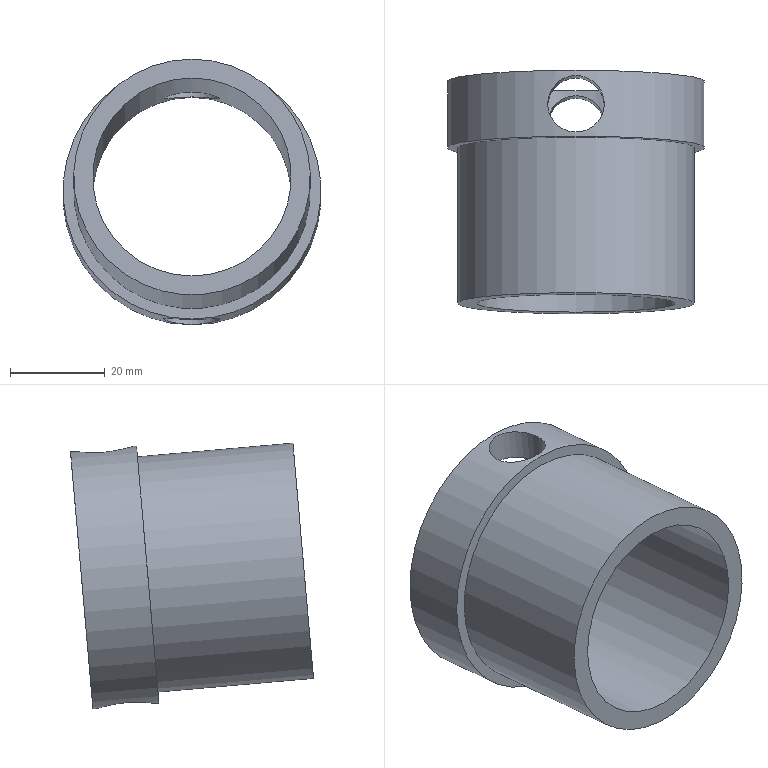Component | NX | SLEEVE | 1 solid | 8 faces | volume 30916 mm3 | cylinder 5 | plane 3 | commonest cylinder face diameters 12 x2 42 x1 54.502 x1 50 x1